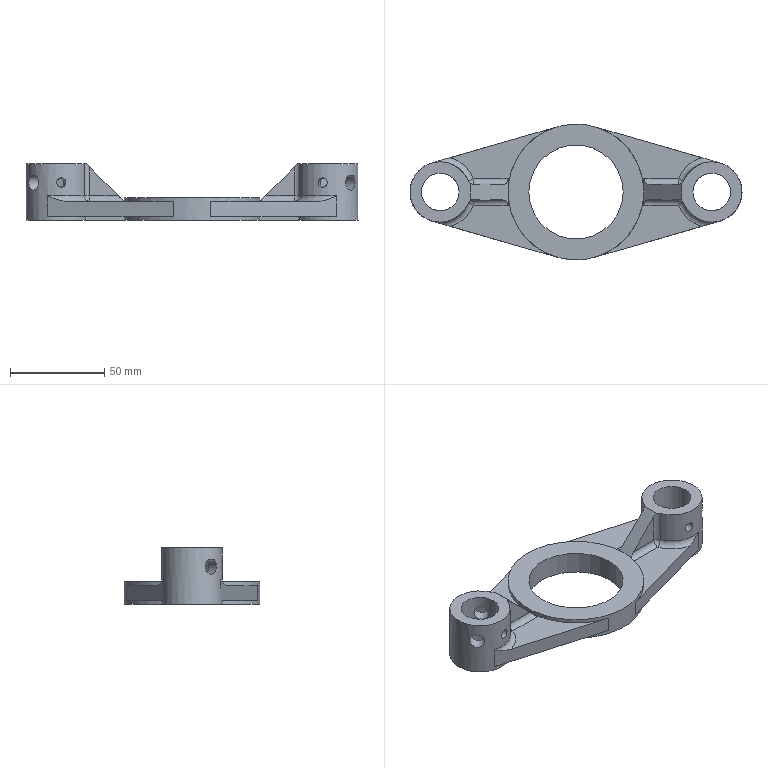Component | NX | WORKPIECE | 1 solid | 56 faces | volume 80747 mm3 | plane 26 | cylinder 22 | sphere 4 | torus 4 | commonest cylinder face diameters 6 x8 32 x4 8 x4 20 x2 5 x2 72 x1 50 x1